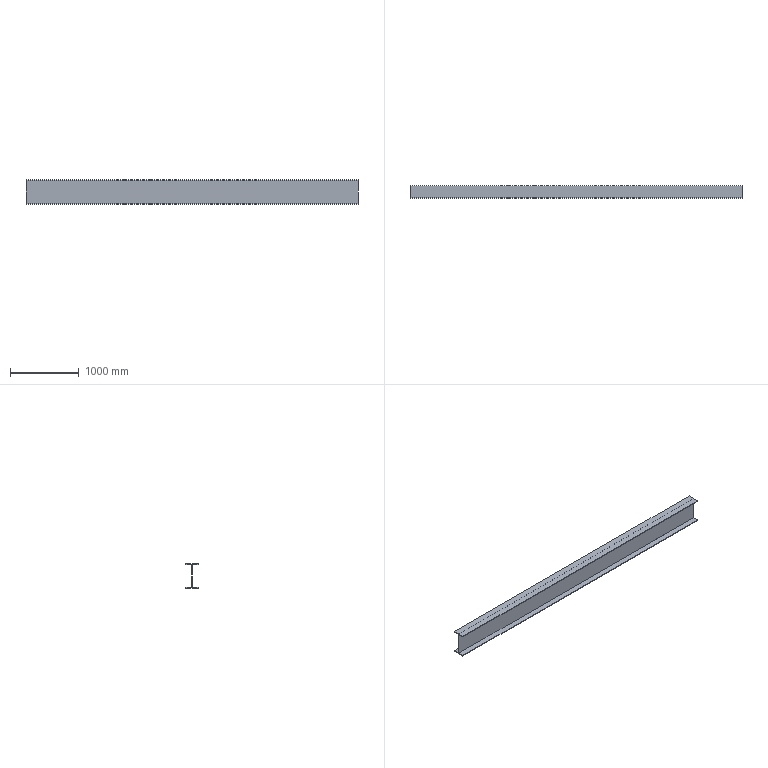Component | NX | ZHIJIA7 | 1 solid | 14 faces | box 4825 x 175 x 350 mm | volume 32810000 mm3 | plane 14
STEP:
#1=CARTESIAN_POINT('',(0.,0.,0.));
#2=DIRECTION('',(0.,0.,1.));
#3=DIRECTION('',(1.,0.,0.));
#4=AXIS2_PLACEMENT_3D('',#1,#2,#3);
#5=CARTESIAN_POINT('',(2412.5,-2807.845,790.));
#6=VERTEX_POINT('',#5);
#7=CARTESIAN_POINT('',(2412.5,-2807.845,800.));
#8=VERTEX_POINT('',#7);
#9=CARTESIAN_POINT('',(2412.5,-2807.845,790.));
#10=DIRECTION('',(0.,-0.,1.));
#11=VECTOR('',#10,1.);
#12=LINE('',#9,#11);
#13=CARTESIAN_POINT('',(-2412.5,-2807.845,790.));
#14=DIRECTION('',(0.,1.,0.));
#15=DIRECTION('',(0.,0.,-1.));
#16=AXIS2_PLACEMENT_3D('',#13,#14,#15);
#17=PLANE('',#16);
#18=CARTESIAN_POINT('',(0.,-4825.));
#19=DIRECTION('',(-1.,0.));
#20=VECTOR('',#19,1.);
#21=LINE('',#18,#20);
#22=(GEOMETRIC_REPRESENTATION_CONTEXT(2)PARAMETRIC_REPRESENTATION_CONTEXT()REPRESENTATION_CONTEXT('',''));
#23=DEFINITIONAL_REPRESENTATION('',(#21),#22);
#24=PCURVE('',#17,#23);
#25=CARTESIAN_POINT('',(2412.5,-2807.845,800.));
#26=DIRECTION('',(-1.,0.,0.));
#27=DIRECTION('',(0.,1.,0.));
#28=AXIS2_PLACEMENT_3D('',#25,#26,#27);
#29=PLANE('',#28);
#30=CARTESIAN_POINT('',(0.,10.));
#31=DIRECTION('',(-0.,-1.));
#32=VECTOR('',#31,1.);
#33=LINE('',#30,#32);
#34=(GEOMETRIC_REPRESENTATION_CONTEXT(2)PARAMETRIC_REPRESENTATION_CONTEXT()REPRESENTATION_CONTEXT('',''));
#35=DEFINITIONAL_REPRESENTATION('',(#33),#34);
#36=PCURVE('',#29,#35);
#37=SURFACE_CURVE('',#12,(#24,#36),.PCURVE_S1.);
#38=EDGE_CURVE('',#6,#8,#37,.T.);
#39=ORIENTED_EDGE('',*,*,#38,.T.);
#40=CARTESIAN_POINT('',(-2412.5,-2807.845,800.));
#41=VERTEX_POINT('',#40);
#42=CARTESIAN_POINT('',(-2412.5,-2807.845,800.));
#43=DIRECTION('',(1.,0.,0.));
#44=VECTOR('',#43,1.);
#45=LINE('',#42,#44);
#46=CARTESIAN_POINT('',(-10.,0.));
#47=DIRECTION('',(0.,-1.));
#48=VECTOR('',#47,1.);
#49=LINE('',#46,#48);
#50=(GEOMETRIC_REPRESENTATION_CONTEXT(2)PARAMETRIC_REPRESENTATION_CONTEXT()REPRESENTATION_CONTEXT('',''));
#51=DEFINITIONAL_REPRESENTATION('',(#49),#50);
#52=PCURVE('',#17,#51);
#53=CARTESIAN_POINT('',(-2412.5,-2807.845,800.));
#54=DIRECTION('',(0.,0.,-1.));
#55=DIRECTION('',(-1.,0.,0.));
#56=AXIS2_PLACEMENT_3D('',#53,#54,#55);
#57=PLANE('',#56);
#58=CARTESIAN_POINT('',(0.,0.));
#59=DIRECTION('',(-1.,0.));
#60=VECTOR('',#59,1.);
#61=LINE('',#58,#60);
#62=(GEOMETRIC_REPRESENTATION_CONTEXT(2)PARAMETRIC_REPRESENTATION_CONTEXT()REPRESENTATION_CONTEXT('',''));
#63=DEFINITIONAL_REPRESENTATION('',(#61),#62);
#64=PCURVE('',#57,#63);
#65=SURFACE_CURVE('',#45,(#52,#64),.PCURVE_S1.);
#66=EDGE_CURVE('',#41,#8,#65,.T.);
#67=ORIENTED_EDGE('',*,*,#66,.F.);
#68=CARTESIAN_POINT('',(-2412.5,-2807.845,790.));
#69=VERTEX_POINT('',#68);
#70=CARTESIAN_POINT('',(-2412.5,-2807.845,790.));
#71=DIRECTION('',(0.,-0.,1.));
#72=VECTOR('',#71,1.);
#73=LINE('',#70,#72);
#74=CARTESIAN_POINT('',(0.,0.));
#75=DIRECTION('',(-1.,0.));
#76=VECTOR('',#75,1.);
#77=LINE('',#74,#76);
#78=(GEOMETRIC_REPRESENTATION_CONTEXT(2)PARAMETRIC_REPRESENTATION_CONTEXT()REPRESENTATION_CONTEXT('',''));
#79=DEFINITIONAL_REPRESENTATION('',(#77),#78);
#80=PCURVE('',#17,#79);
#81=CARTESIAN_POINT('',(-2412.5,-2807.845,800.));
#82=DIRECTION('',(-1.,0.,0.));
#83=DIRECTION('',(0.,1.,0.));
#84=AXIS2_PLACEMENT_3D('',#81,#82,#83);
#85=PLANE('',#84);
#86=CARTESIAN_POINT('',(0.,10.));
#87=DIRECTION('',(-0.,-1.));
#88=VECTOR('',#87,1.);
#89=LINE('',#86,#88);
#90=(GEOMETRIC_REPRESENTATION_CONTEXT(2)PARAMETRIC_REPRESENTATION_CONTEXT()REPRESENTATION_CONTEXT('',''));
#91=DEFINITIONAL_REPRESENTATION('',(#89),#90);
#92=PCURVE('',#85,#91);
#93=SURFACE_CURVE('',#73,(#80,#92),.PCURVE_S1.);
#94=EDGE_CURVE('',#69,#41,#93,.T.);
#95=ORIENTED_EDGE('',*,*,#94,.F.);
#96=CARTESIAN_POINT('',(-2412.5,-2807.845,790.));
#97=DIRECTION('',(1.,0.,0.));
#98=VECTOR('',#97,1.);
#99=LINE('',#96,#98);
#100=CARTESIAN_POINT('',(0.,0.));
#101=DIRECTION('',(0.,-1.));
#102=VECTOR('',#101,1.);
#103=LINE('',#100,#102);
#104=(GEOMETRIC_REPRESENTATION_CONTEXT(2)PARAMETRIC_REPRESENTATION_CONTEXT()REPRESENTATION_CONTEXT('',''));
#105=DEFINITIONAL_REPRESENTATION('',(#103),#104);
#106=PCURVE('',#17,#105);
#107=CARTESIAN_POINT('',(-2412.5,-2725.345,790.));
#108=DIRECTION('',(0.,0.,1.));
#109=DIRECTION('',(1.,0.,0.));
#110=AXIS2_PLACEMENT_3D('',#107,#108,#109);
#111=PLANE('',#110);
#112=CARTESIAN_POINT('',(0.,-82.5));
#113=DIRECTION('',(1.,0.));
#114=VECTOR('',#113,1.);
#115=LINE('',#112,#114);
#116=(GEOMETRIC_REPRESENTATION_CONTEXT(2)PARAMETRIC_REPRESENTATION_CONTEXT()REPRESENTATION_CONTEXT('',''));
#117=DEFINITIONAL_REPRESENTATION('',(#115),#116);
#118=PCURVE('',#111,#117);
#119=SURFACE_CURVE('',#99,(#106,#118),.PCURVE_S1.);
#120=EDGE_CURVE('',#69,#6,#119,.T.);
#121=ORIENTED_EDGE('',*,*,#120,.T.);
#122=EDGE_LOOP('',(#39,#67,#95,#121));
#123=FACE_BOUND('',#122,.T.);
#124=ADVANCED_FACE('',(#123),#17,.F.);
#125=CARTESIAN_POINT('',(2412.5,-2632.845,800.));
#126=VERTEX_POINT('',#125);
#127=CARTESIAN_POINT('',(2412.5,-2807.845,800.));
#128=DIRECTION('',(0.,1.,0.));
#129=VECTOR('',#128,1.);
#130=LINE('',#127,#129);
#131=CARTESIAN_POINT('',(-4825.,0.));
#132=DIRECTION('',(0.,1.));
#133=VECTOR('',#132,1.);
#134=LINE('',#131,#133);
#135=(GEOMETRIC_REPRESENTATION_CONTEXT(2)PARAMETRIC_REPRESENTATION_CONTEXT()REPRESENTATION_CONTEXT('',''));
#136=DEFINITIONAL_REPRESENTATION('',(#134),#135);
#137=PCURVE('',#57,#136);
#138=CARTESIAN_POINT('',(0.,0.));
#139=DIRECTION('',(1.,0.));
#140=VECTOR('',#139,1.);
#141=LINE('',#138,#140);
#142=(GEOMETRIC_REPRESENTATION_CONTEXT(2)PARAMETRIC_REPRESENTATION_CONTEXT()REPRESENTATION_CONTEXT('',''));
#143=DEFINITIONAL_REPRESENTATION('',(#141),#142);
#144=PCURVE('',#29,#143);
#145=SURFACE_CURVE('',#130,(#137,#144),.PCURVE_S1.);
#146=EDGE_CURVE('',#8,#126,#145,.T.);
#147=ORIENTED_EDGE('',*,*,#146,.T.);
#148=CARTESIAN_POINT('',(-2412.5,-2632.845,800.));
#149=VERTEX_POINT('',#148);
#150=CARTESIAN_POINT('',(-2412.5,-2632.845,800.));
#151=DIRECTION('',(1.,0.,0.));
#152=VECTOR('',#151,1.);
#153=LINE('',#150,#152);
#154=CARTESIAN_POINT('',(0.,175.));
#155=DIRECTION('',(-1.,0.));
#156=VECTOR('',#155,1.);
#157=LINE('',#154,#156);
#158=(GEOMETRIC_REPRESENTATION_CONTEXT(2)PARAMETRIC_REPRESENTATION_CONTEXT()REPRESENTATION_CONTEXT('',''));
#159=DEFINITIONAL_REPRESENTATION('',(#157),#158);
#160=PCURVE('',#57,#159);
#161=CARTESIAN_POINT('',(-2412.5,-2632.845,800.));
#162=DIRECTION('',(0.,-1.,-0.));
#163=DIRECTION('',(0.,-0.,1.));
#164=AXIS2_PLACEMENT_3D('',#161,#162,#163);
#165=PLANE('',#164);
#166=CARTESIAN_POINT('',(-0.,0.));
#167=DIRECTION('',(0.,-1.));
#168=VECTOR('',#167,1.);
#169=LINE('',#166,#168);
#170=(GEOMETRIC_REPRESENTATION_CONTEXT(2)PARAMETRIC_REPRESENTATION_CONTEXT()REPRESENTATION_CONTEXT('',''));
#171=DEFINITIONAL_REPRESENTATION('',(#169),#170);
#172=PCURVE('',#165,#171);
#173=SURFACE_CURVE('',#153,(#160,#172),.PCURVE_S1.);
#174=EDGE_CURVE('',#149,#126,#173,.T.);
#175=ORIENTED_EDGE('',*,*,#174,.F.);
#176=CARTESIAN_POINT('',(-2412.5,-2807.845,800.));
#177=DIRECTION('',(0.,1.,0.));
#178=VECTOR('',#177,1.);
#179=LINE('',#176,#178);
#180=CARTESIAN_POINT('',(0.,0.));
#181=DIRECTION('',(0.,1.));
#182=VECTOR('',#181,1.);
#183=LINE('',#180,#182);
#184=(GEOMETRIC_REPRESENTATION_CONTEXT(2)PARAMETRIC_REPRESENTATION_CONTEXT()REPRESENTATION_CONTEXT('',''));
#185=DEFINITIONAL_REPRESENTATION('',(#183),#184);
#186=PCURVE('',#57,#185);
#187=CARTESIAN_POINT('',(0.,0.));
#188=DIRECTION('',(1.,0.));
#189=VECTOR('',#188,1.);
#190=LINE('',#187,#189);
#191=(GEOMETRIC_REPRESENTATION_CONTEXT(2)PARAMETRIC_REPRESENTATION_CONTEXT()REPRESENTATION_CONTEXT('',''));
#192=DEFINITIONAL_REPRESENTATION('',(#190),#191);
#193=PCURVE('',#85,#192);
#194=SURFACE_CURVE('',#179,(#186,#193),.PCURVE_S1.);
#195=EDGE_CURVE('',#41,#149,#194,.T.);
#196=ORIENTED_EDGE('',*,*,#195,.F.);
#197=ORIENTED_EDGE('',*,*,#66,.T.);
#198=EDGE_LOOP('',(#147,#175,#196,#197));
#199=FACE_BOUND('',#198,.T.);
#200=ADVANCED_FACE('',(#199),#57,.F.);
#201=CARTESIAN_POINT('',(2412.5,-2632.845,790.));
#202=VERTEX_POINT('',#201);
#203=CARTESIAN_POINT('',(2412.5,-2632.845,800.));
#204=DIRECTION('',(0.,0.,-1.));
#205=VECTOR('',#204,1.);
#206=LINE('',#203,#205);
#207=CARTESIAN_POINT('',(0.,-4825.));
#208=DIRECTION('',(-1.,0.));
#209=VECTOR('',#208,1.);
#210=LINE('',#207,#209);
#211=(GEOMETRIC_REPRESENTATION_CONTEXT(2)PARAMETRIC_REPRESENTATION_CONTEXT()REPRESENTATION_CONTEXT('',''));
#212=DEFINITIONAL_REPRESENTATION('',(#210),#211);
#213=PCURVE('',#165,#212);
#214=CARTESIAN_POINT('',(175.,-0.));
#215=DIRECTION('',(0.,1.));
#216=VECTOR('',#215,1.);
#217=LINE('',#214,#216);
#218=(GEOMETRIC_REPRESENTATION_CONTEXT(2)PARAMETRIC_REPRESENTATION_CONTEXT()REPRESENTATION_CONTEXT('',''));
#219=DEFINITIONAL_REPRESENTATION('',(#217),#218);
#220=PCURVE('',#29,#219);
#221=SURFACE_CURVE('',#206,(#213,#220),.PCURVE_S1.);
#222=EDGE_CURVE('',#126,#202,#221,.T.);
#223=ORIENTED_EDGE('',*,*,#222,.T.);
#224=CARTESIAN_POINT('',(-2412.5,-2632.845,790.));
#225=VERTEX_POINT('',#224);
#226=CARTESIAN_POINT('',(-2412.5,-2632.845,790.));
#227=DIRECTION('',(1.,0.,0.));
#228=VECTOR('',#227,1.);
#229=LINE('',#226,#228);
#230=CARTESIAN_POINT('',(-10.,0.));
#231=DIRECTION('',(0.,-1.));
#232=VECTOR('',#231,1.);
#233=LINE('',#230,#232);
#234=(GEOMETRIC_REPRESENTATION_CONTEXT(2)PARAMETRIC_REPRESENTATION_CONTEXT()REPRESENTATION_CONTEXT('',''));
#235=DEFINITIONAL_REPRESENTATION('',(#233),#234);
#236=PCURVE('',#165,#235);
#237=CARTESIAN_POINT('',(-2412.5,-2632.845,790.));
#238=DIRECTION('',(0.,0.,1.));
#239=DIRECTION('',(1.,0.,0.));
#240=AXIS2_PLACEMENT_3D('',#237,#238,#239);
#241=PLANE('',#240);
#242=CARTESIAN_POINT('',(0.,0.));
#243=DIRECTION('',(1.,0.));
#244=VECTOR('',#243,1.);
#245=LINE('',#242,#244);
#246=(GEOMETRIC_REPRESENTATION_CONTEXT(2)PARAMETRIC_REPRESENTATION_CONTEXT()REPRESENTATION_CONTEXT('',''));
#247=DEFINITIONAL_REPRESENTATION('',(#245),#246);
#248=PCURVE('',#241,#247);
#249=SURFACE_CURVE('',#229,(#236,#248),.PCURVE_S1.);
#250=EDGE_CURVE('',#225,#202,#249,.T.);
#251=ORIENTED_EDGE('',*,*,#250,.F.);
#252=CARTESIAN_POINT('',(-2412.5,-2632.845,800.));
#253=DIRECTION('',(0.,0.,-1.));
#254=VECTOR('',#253,1.);
#255=LINE('',#252,#254);
#256=CARTESIAN_POINT('',(0.,0.));
#257=DIRECTION('',(-1.,0.));
#258=VECTOR('',#257,1.);
#259=LINE('',#256,#258);
#260=(GEOMETRIC_REPRESENTATION_CONTEXT(2)PARAMETRIC_REPRESENTATION_CONTEXT()REPRESENTATION_CONTEXT('',''));
#261=DEFINITIONAL_REPRESENTATION('',(#259),#260);
#262=PCURVE('',#165,#261);
#263=CARTESIAN_POINT('',(175.,-0.));
#264=DIRECTION('',(0.,1.));
#265=VECTOR('',#264,1.);
#266=LINE('',#263,#265);
#267=(GEOMETRIC_REPRESENTATION_CONTEXT(2)PARAMETRIC_REPRESENTATION_CONTEXT()REPRESENTATION_CONTEXT('',''));
#268=DEFINITIONAL_REPRESENTATION('',(#266),#267);
#269=PCURVE('',#85,#268);
#270=SURFACE_CURVE('',#255,(#262,#269),.PCURVE_S1.);
#271=EDGE_CURVE('',#149,#225,#270,.T.);
#272=ORIENTED_EDGE('',*,*,#271,.F.);
#273=ORIENTED_EDGE('',*,*,#174,.T.);
#274=EDGE_LOOP('',(#223,#251,#272,#273));
#275=FACE_BOUND('',#274,.T.);
#276=ADVANCED_FACE('',(#275),#165,.F.);
#277=CARTESIAN_POINT('',(2412.5,-2715.345,790.));
#278=VERTEX_POINT('',#277);
#279=CARTESIAN_POINT('',(2412.5,-2632.845,790.));
#280=DIRECTION('',(0.,-1.,0.));
#281=VECTOR('',#280,1.);
#282=LINE('',#279,#281);
#283=CARTESIAN_POINT('',(4825.,0.));
#284=DIRECTION('',(0.,-1.));
#285=VECTOR('',#284,1.);
#286=LINE('',#283,#285);
#287=(GEOMETRIC_REPRESENTATION_CONTEXT(2)PARAMETRIC_REPRESENTATION_CONTEXT()REPRESENTATION_CONTEXT('',''));
#288=DEFINITIONAL_REPRESENTATION('',(#286),#287);
#289=PCURVE('',#241,#288);
#290=CARTESIAN_POINT('',(175.,10.));
#291=DIRECTION('',(-1.,0.));
#292=VECTOR('',#291,1.);
#293=LINE('',#290,#292);
#294=(GEOMETRIC_REPRESENTATION_CONTEXT(2)PARAMETRIC_REPRESENTATION_CONTEXT()REPRESENTATION_CONTEXT('',''));
#295=DEFINITIONAL_REPRESENTATION('',(#293),#294);
#296=PCURVE('',#29,#295);
#297=SURFACE_CURVE('',#282,(#289,#296),.PCURVE_S1.);
#298=EDGE_CURVE('',#202,#278,#297,.T.);
#299=ORIENTED_EDGE('',*,*,#298,.T.);
#300=CARTESIAN_POINT('',(-2412.5,-2715.345,790.));
#301=VERTEX_POINT('',#300);
#302=CARTESIAN_POINT('',(-2412.5,-2715.345,790.));
#303=DIRECTION('',(1.,0.,0.));
#304=VECTOR('',#303,1.);
#305=LINE('',#302,#304);
#306=CARTESIAN_POINT('',(0.,-82.5));
#307=DIRECTION('',(1.,0.));
#308=VECTOR('',#307,1.);
#309=LINE('',#306,#308);
#310=(GEOMETRIC_REPRESENTATION_CONTEXT(2)PARAMETRIC_REPRESENTATION_CONTEXT()REPRESENTATION_CONTEXT('',''));
#311=DEFINITIONAL_REPRESENTATION('',(#309),#310);
#312=PCURVE('',#241,#311);
#313=CARTESIAN_POINT('',(-2412.5,-2715.345,790.));
#314=DIRECTION('',(0.,-1.,-0.));
#315=DIRECTION('',(0.,-0.,1.));
#316=AXIS2_PLACEMENT_3D('',#313,#314,#315);
#317=PLANE('',#316);
#318=CARTESIAN_POINT('',(0.,0.));
#319=DIRECTION('',(0.,-1.));
#320=VECTOR('',#319,1.);
#321=LINE('',#318,#320);
#322=(GEOMETRIC_REPRESENTATION_CONTEXT(2)PARAMETRIC_REPRESENTATION_CONTEXT()REPRESENTATION_CONTEXT('',''));
#323=DEFINITIONAL_REPRESENTATION('',(#321),#322);
#324=PCURVE('',#317,#323);
#325=SURFACE_CURVE('',#305,(#312,#324),.PCURVE_S1.);
#326=EDGE_CURVE('',#301,#278,#325,.T.);
#327=ORIENTED_EDGE('',*,*,#326,.F.);
#328=CARTESIAN_POINT('',(-2412.5,-2632.845,790.));
#329=DIRECTION('',(0.,-1.,0.));
#330=VECTOR('',#329,1.);
#331=LINE('',#328,#330);
#332=CARTESIAN_POINT('',(0.,0.));
#333=DIRECTION('',(0.,-1.));
#334=VECTOR('',#333,1.);
#335=LINE('',#332,#334);
#336=(GEOMETRIC_REPRESENTATION_CONTEXT(2)PARAMETRIC_REPRESENTATION_CONTEXT()REPRESENTATION_CONTEXT('',''));
#337=DEFINITIONAL_REPRESENTATION('',(#335),#336);
#338=PCURVE('',#241,#337);
#339=CARTESIAN_POINT('',(175.,10.));
#340=DIRECTION('',(-1.,0.));
#341=VECTOR('',#340,1.);
#342=LINE('',#339,#341);
#343=(GEOMETRIC_REPRESENTATION_CONTEXT(2)PARAMETRIC_REPRESENTATION_CONTEXT()REPRESENTATION_CONTEXT('',''));
#344=DEFINITIONAL_REPRESENTATION('',(#342),#343);
#345=PCURVE('',#85,#344);
#346=SURFACE_CURVE('',#331,(#338,#345),.PCURVE_S1.);
#347=EDGE_CURVE('',#225,#301,#346,.T.);
#348=ORIENTED_EDGE('',*,*,#347,.F.);
#349=ORIENTED_EDGE('',*,*,#250,.T.);
#350=EDGE_LOOP('',(#299,#327,#348,#349));
#351=FACE_BOUND('',#350,.T.);
#352=ADVANCED_FACE('',(#351),#241,.F.);
#353=CARTESIAN_POINT('',(2412.5,-2715.345,460.));
#354=VERTEX_POINT('',#353);
#355=CARTESIAN_POINT('',(2412.5,-2715.345,790.));
#356=DIRECTION('',(0.,0.,-1.));
#357=VECTOR('',#356,1.);
#358=LINE('',#355,#357);
#359=CARTESIAN_POINT('',(0.,-4825.));
#360=DIRECTION('',(-1.,0.));
#361=VECTOR('',#360,1.);
#362=LINE('',#359,#361);
#363=(GEOMETRIC_REPRESENTATION_CONTEXT(2)PARAMETRIC_REPRESENTATION_CONTEXT()REPRESENTATION_CONTEXT('',''));
#364=DEFINITIONAL_REPRESENTATION('',(#362),#363);
#365=PCURVE('',#317,#364);
#366=CARTESIAN_POINT('',(92.5,10.));
#367=DIRECTION('',(0.,1.));
#368=VECTOR('',#367,1.);
#369=LINE('',#366,#368);
#370=(GEOMETRIC_REPRESENTATION_CONTEXT(2)PARAMETRIC_REPRESENTATION_CONTEXT()REPRESENTATION_CONTEXT('',''));
#371=DEFINITIONAL_REPRESENTATION('',(#369),#370);
#372=PCURVE('',#29,#371);
#373=SURFACE_CURVE('',#358,(#365,#372),.PCURVE_S1.);
#374=EDGE_CURVE('',#278,#354,#373,.T.);
#375=ORIENTED_EDGE('',*,*,#374,.T.);
#376=CARTESIAN_POINT('',(-2412.5,-2715.345,460.));
#377=VERTEX_POINT('',#376);
#378=CARTESIAN_POINT('',(-2412.5,-2715.345,460.));
#379=DIRECTION('',(1.,0.,0.));
#380=VECTOR('',#379,1.);
#381=LINE('',#378,#380);
#382=CARTESIAN_POINT('',(-330.,0.));
#383=DIRECTION('',(0.,-1.));
#384=VECTOR('',#383,1.);
#385=LINE('',#382,#384);
#386=(GEOMETRIC_REPRESENTATION_CONTEXT(2)PARAMETRIC_REPRESENTATION_CONTEXT()REPRESENTATION_CONTEXT('',''));
#387=DEFINITIONAL_REPRESENTATION('',(#385),#386);
#388=PCURVE('',#317,#387);
#389=CARTESIAN_POINT('',(-2412.5,-2715.345,460.));
#390=DIRECTION('',(0.,0.,-1.));
#391=DIRECTION('',(-1.,0.,0.));
#392=AXIS2_PLACEMENT_3D('',#389,#390,#391);
#393=PLANE('',#392);
#394=CARTESIAN_POINT('',(0.,0.));
#395=DIRECTION('',(-1.,0.));
#396=VECTOR('',#395,1.);
#397=LINE('',#394,#396);
#398=(GEOMETRIC_REPRESENTATION_CONTEXT(2)PARAMETRIC_REPRESENTATION_CONTEXT()REPRESENTATION_CONTEXT('',''));
#399=DEFINITIONAL_REPRESENTATION('',(#397),#398);
#400=PCURVE('',#393,#399);
#401=SURFACE_CURVE('',#381,(#388,#400),.PCURVE_S1.);
#402=EDGE_CURVE('',#377,#354,#401,.T.);
#403=ORIENTED_EDGE('',*,*,#402,.F.);
#404=CARTESIAN_POINT('',(-2412.5,-2715.345,790.));
#405=DIRECTION('',(0.,0.,-1.));
#406=VECTOR('',#405,1.);
#407=LINE('',#404,#406);
#408=CARTESIAN_POINT('',(0.,0.));
#409=DIRECTION('',(-1.,0.));
#410=VECTOR('',#409,1.);
#411=LINE('',#408,#410);
#412=(GEOMETRIC_REPRESENTATION_CONTEXT(2)PARAMETRIC_REPRESENTATION_CONTEXT()REPRESENTATION_CONTEXT('',''));
#413=DEFINITIONAL_REPRESENTATION('',(#411),#412);
#414=PCURVE('',#317,#413);
#415=CARTESIAN_POINT('',(92.5,10.));
#416=DIRECTION('',(0.,1.));
#417=VECTOR('',#416,1.);
#418=LINE('',#415,#417);
#419=(GEOMETRIC_REPRESENTATION_CONTEXT(2)PARAMETRIC_REPRESENTATION_CONTEXT()REPRESENTATION_CONTEXT('',''));
#420=DEFINITIONAL_REPRESENTATION('',(#418),#419);
#421=PCURVE('',#85,#420);
#422=SURFACE_CURVE('',#407,(#414,#421),.PCURVE_S1.);
#423=EDGE_CURVE('',#301,#377,#422,.T.);
#424=ORIENTED_EDGE('',*,*,#423,.F.);
#425=ORIENTED_EDGE('',*,*,#326,.T.);
#426=EDGE_LOOP('',(#375,#403,#424,#425));
#427=FACE_BOUND('',#426,.T.);
#428=ADVANCED_FACE('',(#427),#317,.F.);
#429=CARTESIAN_POINT('',(2412.5,-2632.845,460.));
#430=VERTEX_POINT('',#429);
#431=CARTESIAN_POINT('',(2412.5,-2715.345,460.));
#432=DIRECTION('',(0.,1.,0.));
#433=VECTOR('',#432,1.);
#434=LINE('',#431,#433);
#435=CARTESIAN_POINT('',(-4825.,0.));
#436=DIRECTION('',(0.,1.));
#437=VECTOR('',#436,1.);
#438=LINE('',#435,#437);
#439=(GEOMETRIC_REPRESENTATION_CONTEXT(2)PARAMETRIC_REPRESENTATION_CONTEXT()REPRESENTATION_CONTEXT('',''));
#440=DEFINITIONAL_REPRESENTATION('',(#438),#439);
#441=PCURVE('',#393,#440);
#442=CARTESIAN_POINT('',(92.5,340.));
#443=DIRECTION('',(1.,0.));
#444=VECTOR('',#443,1.);
#445=LINE('',#442,#444);
#446=(GEOMETRIC_REPRESENTATION_CONTEXT(2)PARAMETRIC_REPRESENTATION_CONTEXT()REPRESENTATION_CONTEXT('',''));
#447=DEFINITIONAL_REPRESENTATION('',(#445),#446);
#448=PCURVE('',#29,#447);
#449=SURFACE_CURVE('',#434,(#441,#448),.PCURVE_S1.);
#450=EDGE_CURVE('',#354,#430,#449,.T.);
#451=ORIENTED_EDGE('',*,*,#450,.T.);
#452=CARTESIAN_POINT('',(-2412.5,-2632.845,460.));
#453=VERTEX_POINT('',#452);
#454=CARTESIAN_POINT('',(-2412.5,-2632.845,460.));
#455=DIRECTION('',(1.,0.,0.));
#456=VECTOR('',#455,1.);
#457=LINE('',#454,#456);
#458=CARTESIAN_POINT('',(0.,82.5));
#459=DIRECTION('',(-1.,0.));
#460=VECTOR('',#459,1.);
#461=LINE('',#458,#460);
#462=(GEOMETRIC_REPRESENTATION_CONTEXT(2)PARAMETRIC_REPRESENTATION_CONTEXT()REPRESENTATION_CONTEXT('',''));
#463=DEFINITIONAL_REPRESENTATION('',(#461),#462);
#464=PCURVE('',#393,#463);
#465=CARTESIAN_POINT('',(-2412.5,-2632.845,460.));
#466=DIRECTION('',(0.,-1.,-0.));
#467=DIRECTION('',(0.,-0.,1.));
#468=AXIS2_PLACEMENT_3D('',#465,#466,#467);
#469=PLANE('',#468);
#470=CARTESIAN_POINT('',(0.,0.));
#471=DIRECTION('',(0.,-1.));
#472=VECTOR('',#471,1.);
#473=LINE('',#470,#472);
#474=(GEOMETRIC_REPRESENTATION_CONTEXT(2)PARAMETRIC_REPRESENTATION_CONTEXT()REPRESENTATION_CONTEXT('',''));
#475=DEFINITIONAL_REPRESENTATION('',(#473),#474);
#476=PCURVE('',#469,#475);
#477=SURFACE_CURVE('',#457,(#464,#476),.PCURVE_S1.);
#478=EDGE_CURVE('',#453,#430,#477,.T.);
#479=ORIENTED_EDGE('',*,*,#478,.F.);
#480=CARTESIAN_POINT('',(-2412.5,-2715.345,460.));
#481=DIRECTION('',(0.,1.,0.));
#482=VECTOR('',#481,1.);
#483=LINE('',#480,#482);
#484=CARTESIAN_POINT('',(0.,0.));
#485=DIRECTION('',(0.,1.));
#486=VECTOR('',#485,1.);
#487=LINE('',#484,#486);
#488=(GEOMETRIC_REPRESENTATION_CONTEXT(2)PARAMETRIC_REPRESENTATION_CONTEXT()REPRESENTATION_CONTEXT('',''));
#489=DEFINITIONAL_REPRESENTATION('',(#487),#488);
#490=PCURVE('',#393,#489);
#491=CARTESIAN_POINT('',(92.5,340.));
#492=DIRECTION('',(1.,0.));
#493=VECTOR('',#492,1.);
#494=LINE('',#491,#493);
#495=(GEOMETRIC_REPRESENTATION_CONTEXT(2)PARAMETRIC_REPRESENTATION_CONTEXT()REPRESENTATION_CONTEXT('',''));
#496=DEFINITIONAL_REPRESENTATION('',(#494),#495);
#497=PCURVE('',#85,#496);
#498=SURFACE_CURVE('',#483,(#490,#497),.PCURVE_S1.);
#499=EDGE_CURVE('',#377,#453,#498,.T.);
#500=ORIENTED_EDGE('',*,*,#499,.F.);
#501=ORIENTED_EDGE('',*,*,#402,.T.);
#502=EDGE_LOOP('',(#451,#479,#500,#501));
#503=FACE_BOUND('',#502,.T.);
#504=ADVANCED_FACE('',(#503),#393,.F.);
#505=CARTESIAN_POINT('',(2412.5,-2632.845,450.));
#506=VERTEX_POINT('',#505);
#507=CARTESIAN_POINT('',(2412.5,-2632.845,460.));
#508=DIRECTION('',(0.,0.,-1.));
#509=VECTOR('',#508,1.);
#510=LINE('',#507,#509);
#511=CARTESIAN_POINT('',(0.,-4825.));
#512=DIRECTION('',(-1.,0.));
#513=VECTOR('',#512,1.);
#514=LINE('',#511,#513);
#515=(GEOMETRIC_REPRESENTATION_CONTEXT(2)PARAMETRIC_REPRESENTATION_CONTEXT()REPRESENTATION_CONTEXT('',''));
#516=DEFINITIONAL_REPRESENTATION('',(#514),#515);
#517=PCURVE('',#469,#516);
#518=CARTESIAN_POINT('',(175.,340.));
#519=DIRECTION('',(0.,1.));
#520=VECTOR('',#519,1.);
#521=LINE('',#518,#520);
#522=(GEOMETRIC_REPRESENTATION_CONTEXT(2)PARAMETRIC_REPRESENTATION_CONTEXT()REPRESENTATION_CONTEXT('',''));
#523=DEFINITIONAL_REPRESENTATION('',(#521),#522);
#524=PCURVE('',#29,#523);
#525=SURFACE_CURVE('',#510,(#517,#524),.PCURVE_S1.);
#526=EDGE_CURVE('',#430,#506,#525,.T.);
#527=ORIENTED_EDGE('',*,*,#526,.T.);
#528=CARTESIAN_POINT('',(-2412.5,-2632.845,450.));
#529=VERTEX_POINT('',#528);
#530=CARTESIAN_POINT('',(-2412.5,-2632.845,450.));
#531=DIRECTION('',(1.,0.,0.));
#532=VECTOR('',#531,1.);
#533=LINE('',#530,#532);
#534=CARTESIAN_POINT('',(-10.,0.));
#535=DIRECTION('',(0.,-1.));
#536=VECTOR('',#535,1.);
#537=LINE('',#534,#536);
#538=(GEOMETRIC_REPRESENTATION_CONTEXT(2)PARAMETRIC_REPRESENTATION_CONTEXT()REPRESENTATION_CONTEXT('',''));
#539=DEFINITIONAL_REPRESENTATION('',(#537),#538);
#540=PCURVE('',#469,#539);
#541=CARTESIAN_POINT('',(-2412.5,-2632.845,450.));
#542=DIRECTION('',(0.,0.,1.));
#543=DIRECTION('',(1.,0.,0.));
#544=AXIS2_PLACEMENT_3D('',#541,#542,#543);
#545=PLANE('',#544);
#546=CARTESIAN_POINT('',(0.,0.));
#547=DIRECTION('',(1.,0.));
#548=VECTOR('',#547,1.);
#549=LINE('',#546,#548);
#550=(GEOMETRIC_REPRESENTATION_CONTEXT(2)PARAMETRIC_REPRESENTATION_CONTEXT()REPRESENTATION_CONTEXT('',''));
#551=DEFINITIONAL_REPRESENTATION('',(#549),#550);
#552=PCURVE('',#545,#551);
#553=SURFACE_CURVE('',#533,(#540,#552),.PCURVE_S1.);
#554=EDGE_CURVE('',#529,#506,#553,.T.);
#555=ORIENTED_EDGE('',*,*,#554,.F.);
#556=CARTESIAN_POINT('',(-2412.5,-2632.845,460.));
#557=DIRECTION('',(0.,0.,-1.));
#558=VECTOR('',#557,1.);
#559=LINE('',#556,#558);
#560=CARTESIAN_POINT('',(0.,0.));
#561=DIRECTION('',(-1.,0.));
#562=VECTOR('',#561,1.);
#563=LINE('',#560,#562);
#564=(GEOMETRIC_REPRESENTATION_CONTEXT(2)PARAMETRIC_REPRESENTATION_CONTEXT()REPRESENTATION_CONTEXT('',''));
#565=DEFINITIONAL_REPRESENTATION('',(#563),#564);
#566=PCURVE('',#469,#565);
#567=CARTESIAN_POINT('',(175.,340.));
#568=DIRECTION('',(0.,1.));
#569=VECTOR('',#568,1.);
#570=LINE('',#567,#569);
#571=(GEOMETRIC_REPRESENTATION_CONTEXT(2)PARAMETRIC_REPRESENTATION_CONTEXT()REPRESENTATION_CONTEXT('',''));
#572=DEFINITIONAL_REPRESENTATION('',(#570),#571);
#573=PCURVE('',#85,#572);
#574=SURFACE_CURVE('',#559,(#566,#573),.PCURVE_S1.);
#575=EDGE_CURVE('',#453,#529,#574,.T.);
#576=ORIENTED_EDGE('',*,*,#575,.F.);
#577=ORIENTED_EDGE('',*,*,#478,.T.);
#578=EDGE_LOOP('',(#527,#555,#576,#577));
#579=FACE_BOUND('',#578,.T.);
#580=ADVANCED_FACE('',(#579),#469,.F.);
#581=CARTESIAN_POINT('',(2412.5,-2807.845,450.));
#582=VERTEX_POINT('',#581);
#583=CARTESIAN_POINT('',(2412.5,-2632.845,450.));
#584=DIRECTION('',(0.,-1.,0.));
#585=VECTOR('',#584,1.);
#586=LINE('',#583,#585);
#587=CARTESIAN_POINT('',(4825.,0.));
#588=DIRECTION('',(0.,-1.));
#589=VECTOR('',#588,1.);
#590=LINE('',#587,#589);
#591=(GEOMETRIC_REPRESENTATION_CONTEXT(2)PARAMETRIC_REPRESENTATION_CONTEXT()REPRESENTATION_CONTEXT('',''));
#592=DEFINITIONAL_REPRESENTATION('',(#590),#591);
#593=PCURVE('',#545,#592);
#594=CARTESIAN_POINT('',(175.,350.));
#595=DIRECTION('',(-1.,0.));
#596=VECTOR('',#595,1.);
#597=LINE('',#594,#596);
#598=(GEOMETRIC_REPRESENTATION_CONTEXT(2)PARAMETRIC_REPRESENTATION_CONTEXT()REPRESENTATION_CONTEXT('',''));
#599=DEFINITIONAL_REPRESENTATION('',(#597),#598);
#600=PCURVE('',#29,#599);
#601=SURFACE_CURVE('',#586,(#593,#600),.PCURVE_S1.);
#602=EDGE_CURVE('',#506,#582,#601,.T.);
#603=ORIENTED_EDGE('',*,*,#602,.T.);
#604=CARTESIAN_POINT('',(-2412.5,-2807.845,450.));
#605=VERTEX_POINT('',#604);
#606=CARTESIAN_POINT('',(-2412.5,-2807.845,450.));
#607=DIRECTION('',(1.,0.,0.));
#608=VECTOR('',#607,1.);
#609=LINE('',#606,#608);
#610=CARTESIAN_POINT('',(0.,-175.));
#611=DIRECTION('',(1.,0.));
#612=VECTOR('',#611,1.);
#613=LINE('',#610,#612);
#614=(GEOMETRIC_REPRESENTATION_CONTEXT(2)PARAMETRIC_REPRESENTATION_CONTEXT()REPRESENTATION_CONTEXT('',''));
#615=DEFINITIONAL_REPRESENTATION('',(#613),#614);
#616=PCURVE('',#545,#615);
#617=CARTESIAN_POINT('',(-2412.5,-2807.845,450.));
#618=DIRECTION('',(0.,1.,0.));
#619=DIRECTION('',(0.,0.,-1.));
#620=AXIS2_PLACEMENT_3D('',#617,#618,#619);
#621=PLANE('',#620);
#622=CARTESIAN_POINT('',(0.,0.));
#623=DIRECTION('',(0.,-1.));
#624=VECTOR('',#623,1.);
#625=LINE('',#622,#624);
#626=(GEOMETRIC_REPRESENTATION_CONTEXT(2)PARAMETRIC_REPRESENTATION_CONTEXT()REPRESENTATION_CONTEXT('',''));
#627=DEFINITIONAL_REPRESENTATION('',(#625),#626);
#628=PCURVE('',#621,#627);
#629=SURFACE_CURVE('',#609,(#616,#628),.PCURVE_S1.);
#630=EDGE_CURVE('',#605,#582,#629,.T.);
#631=ORIENTED_EDGE('',*,*,#630,.F.);
#632=CARTESIAN_POINT('',(-2412.5,-2632.845,450.));
#633=DIRECTION('',(0.,-1.,0.));
#634=VECTOR('',#633,1.);
#635=LINE('',#632,#634);
#636=CARTESIAN_POINT('',(0.,0.));
#637=DIRECTION('',(0.,-1.));
#638=VECTOR('',#637,1.);
#639=LINE('',#636,#638);
#640=(GEOMETRIC_REPRESENTATION_CONTEXT(2)PARAMETRIC_REPRESENTATION_CONTEXT()REPRESENTATION_CONTEXT('',''));
#641=DEFINITIONAL_REPRESENTATION('',(#639),#640);
#642=PCURVE('',#545,#641);
#643=CARTESIAN_POINT('',(175.,350.));
#644=DIRECTION('',(-1.,0.));
#645=VECTOR('',#644,1.);
#646=LINE('',#643,#645);
#647=(GEOMETRIC_REPRESENTATION_CONTEXT(2)PARAMETRIC_REPRESENTATION_CONTEXT()REPRESENTATION_CONTEXT('',''));
#648=DEFINITIONAL_REPRESENTATION('',(#646),#647);
#649=PCURVE('',#85,#648);
#650=SURFACE_CURVE('',#635,(#642,#649),.PCURVE_S1.);
#651=EDGE_CURVE('',#529,#605,#650,.T.);
#652=ORIENTED_EDGE('',*,*,#651,.F.);
#653=ORIENTED_EDGE('',*,*,#554,.T.);
#654=EDGE_LOOP('',(#603,#631,#652,#653));
#655=FACE_BOUND('',#654,.T.);
#656=ADVANCED_FACE('',(#655),#545,.F.);
#657=CARTESIAN_POINT('',(2412.5,-2807.845,460.));
#658=VERTEX_POINT('',#657);
#659=CARTESIAN_POINT('',(2412.5,-2807.845,450.));
#660=DIRECTION('',(0.,-0.,1.));
#661=VECTOR('',#660,1.);
#662=LINE('',#659,#661);
#663=CARTESIAN_POINT('',(0.,-4825.));
#664=DIRECTION('',(-1.,0.));
#665=VECTOR('',#664,1.);
#666=LINE('',#663,#665);
#667=(GEOMETRIC_REPRESENTATION_CONTEXT(2)PARAMETRIC_REPRESENTATION_CONTEXT()REPRESENTATION_CONTEXT('',''));
#668=DEFINITIONAL_REPRESENTATION('',(#666),#667);
#669=PCURVE('',#621,#668);
#670=CARTESIAN_POINT('',(0.,350.));
#671=DIRECTION('',(-0.,-1.));
#672=VECTOR('',#671,1.);
#673=LINE('',#670,#672);
#674=(GEOMETRIC_REPRESENTATION_CONTEXT(2)PARAMETRIC_REPRESENTATION_CONTEXT()REPRESENTATION_CONTEXT('',''));
#675=DEFINITIONAL_REPRESENTATION('',(#673),#674);
#676=PCURVE('',#29,#675);
#677=SURFACE_CURVE('',#662,(#669,#676),.PCURVE_S1.);
#678=EDGE_CURVE('',#582,#658,#677,.T.);
#679=ORIENTED_EDGE('',*,*,#678,.T.);
#680=CARTESIAN_POINT('',(-2412.5,-2807.845,460.));
#681=VERTEX_POINT('',#680);
#682=CARTESIAN_POINT('',(-2412.5,-2807.845,460.));
#683=DIRECTION('',(1.,0.,0.));
#684=VECTOR('',#683,1.);
#685=LINE('',#682,#684);
#686=CARTESIAN_POINT('',(-10.,0.));
#687=DIRECTION('',(0.,-1.));
#688=VECTOR('',#687,1.);
#689=LINE('',#686,#688);
#690=(GEOMETRIC_REPRESENTATION_CONTEXT(2)PARAMETRIC_REPRESENTATION_CONTEXT()REPRESENTATION_CONTEXT('',''));
#691=DEFINITIONAL_REPRESENTATION('',(#689),#690);
#692=PCURVE('',#621,#691);
#693=CARTESIAN_POINT('',(-2412.5,-2807.845,460.));
#694=DIRECTION('',(0.,0.,-1.));
#695=DIRECTION('',(-1.,0.,0.));
#696=AXIS2_PLACEMENT_3D('',#693,#694,#695);
#697=PLANE('',#696);
#698=CARTESIAN_POINT('',(0.,0.));
#699=DIRECTION('',(-1.,0.));
#700=VECTOR('',#699,1.);
#701=LINE('',#698,#700);
#702=(GEOMETRIC_REPRESENTATION_CONTEXT(2)PARAMETRIC_REPRESENTATION_CONTEXT()REPRESENTATION_CONTEXT('',''));
#703=DEFINITIONAL_REPRESENTATION('',(#701),#702);
#704=PCURVE('',#697,#703);
#705=SURFACE_CURVE('',#685,(#692,#704),.PCURVE_S1.);
#706=EDGE_CURVE('',#681,#658,#705,.T.);
#707=ORIENTED_EDGE('',*,*,#706,.F.);
#708=CARTESIAN_POINT('',(-2412.5,-2807.845,450.));
#709=DIRECTION('',(0.,-0.,1.));
#710=VECTOR('',#709,1.);
#711=LINE('',#708,#710);
#712=CARTESIAN_POINT('',(0.,0.));
#713=DIRECTION('',(-1.,0.));
#714=VECTOR('',#713,1.);
#715=LINE('',#712,#714);
#716=(GEOMETRIC_REPRESENTATION_CONTEXT(2)PARAMETRIC_REPRESENTATION_CONTEXT()REPRESENTATION_CONTEXT('',''));
#717=DEFINITIONAL_REPRESENTATION('',(#715),#716);
#718=PCURVE('',#621,#717);
#719=CARTESIAN_POINT('',(0.,350.));
#720=DIRECTION('',(-0.,-1.));
#721=VECTOR('',#720,1.);
#722=LINE('',#719,#721);
#723=(GEOMETRIC_REPRESENTATION_CONTEXT(2)PARAMETRIC_REPRESENTATION_CONTEXT()REPRESENTATION_CONTEXT('',''));
#724=DEFINITIONAL_REPRESENTATION('',(#722),#723);
#725=PCURVE('',#85,#724);
#726=SURFACE_CURVE('',#711,(#718,#725),.PCURVE_S1.);
#727=EDGE_CURVE('',#605,#681,#726,.T.);
#728=ORIENTED_EDGE('',*,*,#727,.F.);
#729=ORIENTED_EDGE('',*,*,#630,.T.);
#730=EDGE_LOOP('',(#679,#707,#728,#729));
#731=FACE_BOUND('',#730,.T.);
#732=ADVANCED_FACE('',(#731),#621,.F.);
#733=CARTESIAN_POINT('',(2412.5,-2725.345,460.));
#734=VERTEX_POINT('',#733);
#735=CARTESIAN_POINT('',(2412.5,-2807.845,460.));
#736=DIRECTION('',(0.,1.,0.));
#737=VECTOR('',#736,1.);
#738=LINE('',#735,#737);
#739=CARTESIAN_POINT('',(-4825.,0.));
#740=DIRECTION('',(0.,1.));
#741=VECTOR('',#740,1.);
#742=LINE('',#739,#741);
#743=(GEOMETRIC_REPRESENTATION_CONTEXT(2)PARAMETRIC_REPRESENTATION_CONTEXT()REPRESENTATION_CONTEXT('',''));
#744=DEFINITIONAL_REPRESENTATION('',(#742),#743);
#745=PCURVE('',#697,#744);
#746=CARTESIAN_POINT('',(0.,340.));
#747=DIRECTION('',(1.,0.));
#748=VECTOR('',#747,1.);
#749=LINE('',#746,#748);
#750=(GEOMETRIC_REPRESENTATION_CONTEXT(2)PARAMETRIC_REPRESENTATION_CONTEXT()REPRESENTATION_CONTEXT('',''));
#751=DEFINITIONAL_REPRESENTATION('',(#749),#750);
#752=PCURVE('',#29,#751);
#753=SURFACE_CURVE('',#738,(#745,#752),.PCURVE_S1.);
#754=EDGE_CURVE('',#658,#734,#753,.T.);
#755=ORIENTED_EDGE('',*,*,#754,.T.);
#756=CARTESIAN_POINT('',(-2412.5,-2725.345,460.));
#757=VERTEX_POINT('',#756);
#758=CARTESIAN_POINT('',(-2412.5,-2725.345,460.));
#759=DIRECTION('',(1.,0.,0.));
#760=VECTOR('',#759,1.);
#761=LINE('',#758,#760);
#762=CARTESIAN_POINT('',(0.,82.5));
#763=DIRECTION('',(-1.,0.));
#764=VECTOR('',#763,1.);
#765=LINE('',#762,#764);
#766=(GEOMETRIC_REPRESENTATION_CONTEXT(2)PARAMETRIC_REPRESENTATION_CONTEXT()REPRESENTATION_CONTEXT('',''));
#767=DEFINITIONAL_REPRESENTATION('',(#765),#766);
#768=PCURVE('',#697,#767);
#769=CARTESIAN_POINT('',(-2412.5,-2725.345,460.));
#770=DIRECTION('',(0.,1.,0.));
#771=DIRECTION('',(0.,0.,-1.));
#772=AXIS2_PLACEMENT_3D('',#769,#770,#771);
#773=PLANE('',#772);
#774=CARTESIAN_POINT('',(0.,0.));
#775=DIRECTION('',(0.,-1.));
#776=VECTOR('',#775,1.);
#777=LINE('',#774,#776);
#778=(GEOMETRIC_REPRESENTATION_CONTEXT(2)PARAMETRIC_REPRESENTATION_CONTEXT()REPRESENTATION_CONTEXT('',''));
#779=DEFINITIONAL_REPRESENTATION('',(#777),#778);
#780=PCURVE('',#773,#779);
#781=SURFACE_CURVE('',#761,(#768,#780),.PCURVE_S1.);
#782=EDGE_CURVE('',#757,#734,#781,.T.);
#783=ORIENTED_EDGE('',*,*,#782,.F.);
#784=CARTESIAN_POINT('',(-2412.5,-2807.845,460.));
#785=DIRECTION('',(0.,1.,0.));
#786=VECTOR('',#785,1.);
#787=LINE('',#784,#786);
#788=CARTESIAN_POINT('',(0.,0.));
#789=DIRECTION('',(0.,1.));
#790=VECTOR('',#789,1.);
#791=LINE('',#788,#790);
#792=(GEOMETRIC_REPRESENTATION_CONTEXT(2)PARAMETRIC_REPRESENTATION_CONTEXT()REPRESENTATION_CONTEXT('',''));
#793=DEFINITIONAL_REPRESENTATION('',(#791),#792);
#794=PCURVE('',#697,#793);
#795=CARTESIAN_POINT('',(0.,340.));
#796=DIRECTION('',(1.,0.));
#797=VECTOR('',#796,1.);
#798=LINE('',#795,#797);
#799=(GEOMETRIC_REPRESENTATION_CONTEXT(2)PARAMETRIC_REPRESENTATION_CONTEXT()REPRESENTATION_CONTEXT('',''));
#800=DEFINITIONAL_REPRESENTATION('',(#798),#799);
#801=PCURVE('',#85,#800);
#802=SURFACE_CURVE('',#787,(#794,#801),.PCURVE_S1.);
#803=EDGE_CURVE('',#681,#757,#802,.T.);
#804=ORIENTED_EDGE('',*,*,#803,.F.);
#805=ORIENTED_EDGE('',*,*,#706,.T.);
#806=EDGE_LOOP('',(#755,#783,#804,#805));
#807=FACE_BOUND('',#806,.T.);
#808=ADVANCED_FACE('',(#807),#697,.F.);
#809=CARTESIAN_POINT('',(2412.5,-2725.345,790.));
#810=VERTEX_POINT('',#809);
#811=CARTESIAN_POINT('',(2412.5,-2725.345,460.));
#812=DIRECTION('',(0.,-0.,1.));
#813=VECTOR('',#812,1.);
#814=LINE('',#811,#813);
#815=CARTESIAN_POINT('',(0.,-4825.));
#816=DIRECTION('',(-1.,0.));
#817=VECTOR('',#816,1.);
#818=LINE('',#815,#817);
#819=(GEOMETRIC_REPRESENTATION_CONTEXT(2)PARAMETRIC_REPRESENTATION_CONTEXT()REPRESENTATION_CONTEXT('',''));
#820=DEFINITIONAL_REPRESENTATION('',(#818),#819);
#821=PCURVE('',#773,#820);
#822=CARTESIAN_POINT('',(82.5,340.));
#823=DIRECTION('',(-0.,-1.));
#824=VECTOR('',#823,1.);
#825=LINE('',#822,#824);
#826=(GEOMETRIC_REPRESENTATION_CONTEXT(2)PARAMETRIC_REPRESENTATION_CONTEXT()REPRESENTATION_CONTEXT('',''));
#827=DEFINITIONAL_REPRESENTATION('',(#825),#826);
#828=PCURVE('',#29,#827);
#829=SURFACE_CURVE('',#814,(#821,#828),.PCURVE_S1.);
#830=EDGE_CURVE('',#734,#810,#829,.T.);
#831=ORIENTED_EDGE('',*,*,#830,.T.);
#832=CARTESIAN_POINT('',(-2412.5,-2725.345,790.));
#833=VERTEX_POINT('',#832);
#834=CARTESIAN_POINT('',(-2412.5,-2725.345,790.));
#835=DIRECTION('',(1.,0.,0.));
#836=VECTOR('',#835,1.);
#837=LINE('',#834,#836);
#838=CARTESIAN_POINT('',(-330.,0.));
#839=DIRECTION('',(0.,-1.));
#840=VECTOR('',#839,1.);
#841=LINE('',#838,#840);
#842=(GEOMETRIC_REPRESENTATION_CONTEXT(2)PARAMETRIC_REPRESENTATION_CONTEXT()REPRESENTATION_CONTEXT('',''));
#843=DEFINITIONAL_REPRESENTATION('',(#841),#842);
#844=PCURVE('',#773,#843);
#845=CARTESIAN_POINT('',(0.,0.));
#846=DIRECTION('',(1.,0.));
#847=VECTOR('',#846,1.);
#848=LINE('',#845,#847);
#849=(GEOMETRIC_REPRESENTATION_CONTEXT(2)PARAMETRIC_REPRESENTATION_CONTEXT()REPRESENTATION_CONTEXT('',''));
#850=DEFINITIONAL_REPRESENTATION('',(#848),#849);
#851=PCURVE('',#111,#850);
#852=SURFACE_CURVE('',#837,(#844,#851),.PCURVE_S1.);
#853=EDGE_CURVE('',#833,#810,#852,.T.);
#854=ORIENTED_EDGE('',*,*,#853,.F.);
#855=CARTESIAN_POINT('',(-2412.5,-2725.345,460.));
#856=DIRECTION('',(0.,-0.,1.));
#857=VECTOR('',#856,1.);
#858=LINE('',#855,#857);
#859=CARTESIAN_POINT('',(0.,0.));
#860=DIRECTION('',(-1.,0.));
#861=VECTOR('',#860,1.);
#862=LINE('',#859,#861);
#863=(GEOMETRIC_REPRESENTATION_CONTEXT(2)PARAMETRIC_REPRESENTATION_CONTEXT()REPRESENTATION_CONTEXT('',''));
#864=DEFINITIONAL_REPRESENTATION('',(#862),#863);
#865=PCURVE('',#773,#864);
#866=CARTESIAN_POINT('',(82.5,340.));
#867=DIRECTION('',(-0.,-1.));
#868=VECTOR('',#867,1.);
#869=LINE('',#866,#868);
#870=(GEOMETRIC_REPRESENTATION_CONTEXT(2)PARAMETRIC_REPRESENTATION_CONTEXT()REPRESENTATION_CONTEXT('',''));
#871=DEFINITIONAL_REPRESENTATION('',(#869),#870);
#872=PCURVE('',#85,#871);
#873=SURFACE_CURVE('',#858,(#865,#872),.PCURVE_S1.);
#874=EDGE_CURVE('',#757,#833,#873,.T.);
#875=ORIENTED_EDGE('',*,*,#874,.F.);
#876=ORIENTED_EDGE('',*,*,#782,.T.);
#877=EDGE_LOOP('',(#831,#854,#875,#876));
#878=FACE_BOUND('',#877,.T.);
#879=ADVANCED_FACE('',(#878),#773,.F.);
#880=CARTESIAN_POINT('',(2412.5,-2725.345,790.));
#881=DIRECTION('',(0.,-1.,0.));
#882=VECTOR('',#881,1.);
#883=LINE('',#880,#882);
#884=CARTESIAN_POINT('',(4825.,0.));
#885=DIRECTION('',(0.,-1.));
#886=VECTOR('',#885,1.);
#887=LINE('',#884,#886);
#888=(GEOMETRIC_REPRESENTATION_CONTEXT(2)PARAMETRIC_REPRESENTATION_CONTEXT()REPRESENTATION_CONTEXT('',''));
#889=DEFINITIONAL_REPRESENTATION('',(#887),#888);
#890=PCURVE('',#111,#889);
#891=CARTESIAN_POINT('',(82.5,10.));
#892=DIRECTION('',(-1.,0.));
#893=VECTOR('',#892,1.);
#894=LINE('',#891,#893);
#895=(GEOMETRIC_REPRESENTATION_CONTEXT(2)PARAMETRIC_REPRESENTATION_CONTEXT()REPRESENTATION_CONTEXT('',''));
#896=DEFINITIONAL_REPRESENTATION('',(#894),#895);
#897=PCURVE('',#29,#896);
#898=SURFACE_CURVE('',#883,(#890,#897),.PCURVE_S1.);
#899=EDGE_CURVE('',#810,#6,#898,.T.);
#900=ORIENTED_EDGE('',*,*,#899,.T.);
#901=ORIENTED_EDGE('',*,*,#120,.F.);
#902=CARTESIAN_POINT('',(-2412.5,-2725.345,790.));
#903=DIRECTION('',(0.,-1.,0.));
#904=VECTOR('',#903,1.);
#905=LINE('',#902,#904);
#906=CARTESIAN_POINT('',(0.,0.));
#907=DIRECTION('',(0.,-1.));
#908=VECTOR('',#907,1.);
#909=LINE('',#906,#908);
#910=(GEOMETRIC_REPRESENTATION_CONTEXT(2)PARAMETRIC_REPRESENTATION_CONTEXT()REPRESENTATION_CONTEXT('',''));
#911=DEFINITIONAL_REPRESENTATION('',(#909),#910);
#912=PCURVE('',#111,#911);
#913=CARTESIAN_POINT('',(82.5,10.));
#914=DIRECTION('',(-1.,0.));
#915=VECTOR('',#914,1.);
#916=LINE('',#913,#915);
#917=(GEOMETRIC_REPRESENTATION_CONTEXT(2)PARAMETRIC_REPRESENTATION_CONTEXT()REPRESENTATION_CONTEXT('',''));
#918=DEFINITIONAL_REPRESENTATION('',(#916),#917);
#919=PCURVE('',#85,#918);
#920=SURFACE_CURVE('',#905,(#912,#919),.PCURVE_S1.);
#921=EDGE_CURVE('',#833,#69,#920,.T.);
#922=ORIENTED_EDGE('',*,*,#921,.F.);
#923=ORIENTED_EDGE('',*,*,#853,.T.);
#924=EDGE_LOOP('',(#900,#901,#922,#923));
#925=FACE_BOUND('',#924,.T.);
#926=ADVANCED_FACE('',(#925),#111,.F.);
#927=ORIENTED_EDGE('',*,*,#94,.T.);
#928=ORIENTED_EDGE('',*,*,#195,.T.);
#929=ORIENTED_EDGE('',*,*,#271,.T.);
#930=ORIENTED_EDGE('',*,*,#347,.T.);
#931=ORIENTED_EDGE('',*,*,#423,.T.);
#932=ORIENTED_EDGE('',*,*,#499,.T.);
#933=ORIENTED_EDGE('',*,*,#575,.T.);
#934=ORIENTED_EDGE('',*,*,#651,.T.);
#935=ORIENTED_EDGE('',*,*,#727,.T.);
#936=ORIENTED_EDGE('',*,*,#803,.T.);
#937=ORIENTED_EDGE('',*,*,#874,.T.);
#938=ORIENTED_EDGE('',*,*,#921,.T.);
#939=EDGE_LOOP('',(#927,#928,#929,#930,#931,#932,#933,#934,#935,#936,#937,#938));
#940=FACE_BOUND('',#939,.T.);
#941=ADVANCED_FACE('',(#940),#85,.T.);
#942=ORIENTED_EDGE('',*,*,#38,.F.);
#943=ORIENTED_EDGE('',*,*,#899,.F.);
#944=ORIENTED_EDGE('',*,*,#830,.F.);
#945=ORIENTED_EDGE('',*,*,#754,.F.);
#946=ORIENTED_EDGE('',*,*,#678,.F.);
#947=ORIENTED_EDGE('',*,*,#602,.F.);
#948=ORIENTED_EDGE('',*,*,#526,.F.);
#949=ORIENTED_EDGE('',*,*,#450,.F.);
#950=ORIENTED_EDGE('',*,*,#374,.F.);
#951=ORIENTED_EDGE('',*,*,#298,.F.);
#952=ORIENTED_EDGE('',*,*,#222,.F.);
#953=ORIENTED_EDGE('',*,*,#146,.F.);
#954=EDGE_LOOP('',(#942,#943,#944,#945,#946,#947,#948,#949,#950,#951,#952,#953));
#955=FACE_BOUND('',#954,.T.);
#956=ADVANCED_FACE('',(#955),#29,.F.);
#957=CLOSED_SHELL('',(#124,#200,#276,#352,#428,#504,#580,#656,#732,#808,#879,#926,#941,#956));
#958=MANIFOLD_SOLID_BREP('',#957);
#959=(LENGTH_UNIT()NAMED_UNIT(*)SI_UNIT(.MILLI.,.METRE.));
#960=UNCERTAINTY_MEASURE_WITH_UNIT(LENGTH_MEASURE(0.0000001),#959,'','');
#961=(NAMED_UNIT(*)PLANE_ANGLE_UNIT()SI_UNIT($,.RADIAN.));
#962=(NAMED_UNIT(*)SI_UNIT($,.STERADIAN.)SOLID_ANGLE_UNIT());
#963=(GEOMETRIC_REPRESENTATION_CONTEXT(3)GLOBAL_UNCERTAINTY_ASSIGNED_CONTEXT((#960))GLOBAL_UNIT_ASSIGNED_CONTEXT((#959,#961,#962))REPRESENTATION_CONTEXT('',''));
#964=ADVANCED_BREP_SHAPE_REPRESENTATION('',(#4,#958),#963);